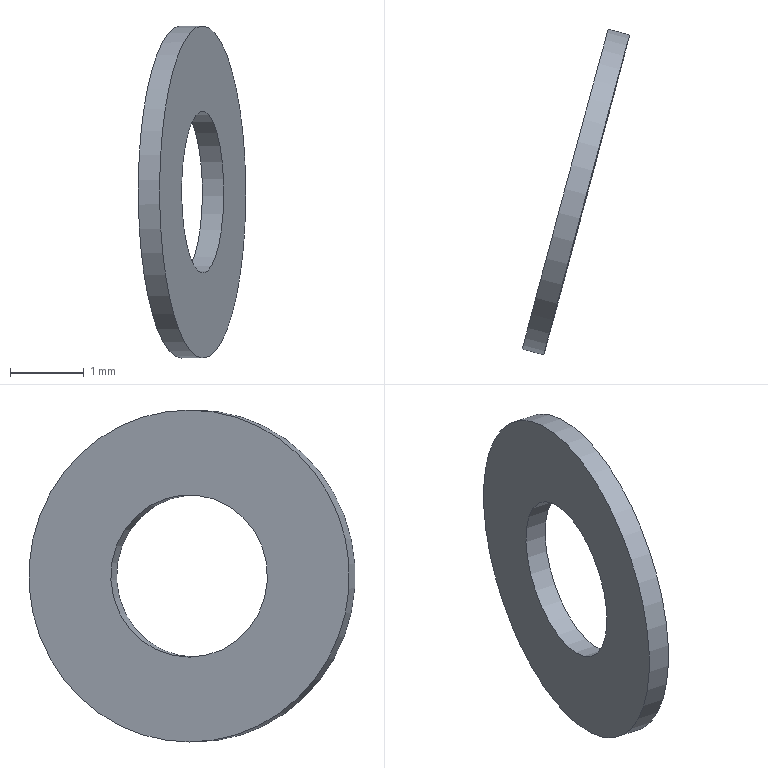Component | NX | GB-T848-2002_M2 | 1 solid | 4 faces | box 1.46 x 4.42 x 4.5 mm | volume 4 mm3 | cylinder 2 | plane 2 | commonest cylinder face diameters 4.5 x1 2.2 x1
STEP:
#1=CARTESIAN_POINT('',(0.,0.,0.));
#2=DIRECTION('',(0.,0.,1.));
#3=DIRECTION('',(1.,0.,0.));
#4=AXIS2_PLACEMENT_3D('',#1,#2,#3);
#5=CARTESIAN_POINT('',(52.266,-56.588,80.689));
#6=VERTEX_POINT('',#5);
#7=CARTESIAN_POINT('',(52.262,-56.588,82.939));
#8=DIRECTION('',(0.9657,-0.2595,0.001964));
#9=DIRECTION('',(0.002034,0.,-1.));
#10=AXIS2_PLACEMENT_3D('',#7,#8,#9);
#11=CIRCLE('',#10,2.25);
#12=CARTESIAN_POINT('',(52.262,-56.588,82.939));
#13=DIRECTION('',(-0.9657,0.2595,-0.001964));
#14=DIRECTION('',(-0.002034,-0.,1.));
#15=AXIS2_PLACEMENT_3D('',#12,#13,#14);
#16=CYLINDRICAL_SURFACE('',#15,2.25);
#17=CARTESIAN_POINT('',(9.425,0.));
#18=DIRECTION('',(-1.,0.));
#19=VECTOR('',#18,1.);
#20=LINE('',#17,#19);
#21=(GEOMETRIC_REPRESENTATION_CONTEXT(2)PARAMETRIC_REPRESENTATION_CONTEXT()REPRESENTATION_CONTEXT('',''));
#22=DEFINITIONAL_REPRESENTATION('',(#20),#21);
#23=PCURVE('',#16,#22);
#24=CARTESIAN_POINT('',(52.262,-56.588,82.939));
#25=DIRECTION('',(0.9657,-0.2595,0.001964));
#26=DIRECTION('',(0.002034,0.,-1.));
#27=AXIS2_PLACEMENT_3D('',#24,#25,#26);
#28=PLANE('',#27);
#29=CARTESIAN_POINT('',(0.,0.));
#30=DIRECTION('',(1.,0.));
#31=AXIS2_PLACEMENT_2D('',#29,#30);
#32=CIRCLE('',#31,2.25);
#33=(GEOMETRIC_REPRESENTATION_CONTEXT(2)PARAMETRIC_REPRESENTATION_CONTEXT()REPRESENTATION_CONTEXT('',''));
#34=DEFINITIONAL_REPRESENTATION('',(#32),#33);
#35=PCURVE('',#28,#34);
#36=SURFACE_CURVE('',#11,(#23,#35),.PCURVE_S1.);
#37=EDGE_CURVE('',#6,#6,#36,.T.);
#38=ORIENTED_EDGE('',*,*,#37,.F.);
#39=CARTESIAN_POINT('',(51.977,-56.51,80.688));
#40=VERTEX_POINT('',#39);
#41=CARTESIAN_POINT('',(52.266,-56.588,80.689));
#42=CARTESIAN_POINT('',(51.977,-56.51,80.688));
#43=B_SPLINE_CURVE_WITH_KNOTS('',1,(#41,#42),.UNSPECIFIED.,.F.,.F.,(2,2),(0.,0.3),.PIECEWISE_BEZIER_KNOTS.);
#44=CARTESIAN_POINT('',(9.425,0.));
#45=DIRECTION('',(0.,1.));
#46=VECTOR('',#45,1.);
#47=LINE('',#44,#46);
#48=(GEOMETRIC_REPRESENTATION_CONTEXT(2)PARAMETRIC_REPRESENTATION_CONTEXT()REPRESENTATION_CONTEXT('',''));
#49=DEFINITIONAL_REPRESENTATION('',(#47),#48);
#50=PCURVE('',#16,#49);
#51=CARTESIAN_POINT('',(3.142,0.));
#52=DIRECTION('',(0.,1.));
#53=VECTOR('',#52,1.);
#54=LINE('',#51,#53);
#55=(GEOMETRIC_REPRESENTATION_CONTEXT(2)PARAMETRIC_REPRESENTATION_CONTEXT()REPRESENTATION_CONTEXT('',''));
#56=DEFINITIONAL_REPRESENTATION('',(#54),#55);
#57=PCURVE('',#16,#56);
#58=SEAM_CURVE('',#43,(#50,#57),.PCURVE_S1.);
#59=EDGE_CURVE('',#6,#40,#58,.T.);
#60=ORIENTED_EDGE('',*,*,#59,.T.);
#61=CARTESIAN_POINT('',(51.972,-56.51,82.938));
#62=DIRECTION('',(0.9657,-0.2595,0.001964));
#63=DIRECTION('',(0.002034,0.,-1.));
#64=AXIS2_PLACEMENT_3D('',#61,#62,#63);
#65=CIRCLE('',#64,2.25);
#66=CARTESIAN_POINT('',(9.425,0.3));
#67=DIRECTION('',(-1.,0.));
#68=VECTOR('',#67,1.);
#69=LINE('',#66,#68);
#70=(GEOMETRIC_REPRESENTATION_CONTEXT(2)PARAMETRIC_REPRESENTATION_CONTEXT()REPRESENTATION_CONTEXT('',''));
#71=DEFINITIONAL_REPRESENTATION('',(#69),#70);
#72=PCURVE('',#16,#71);
#73=CARTESIAN_POINT('',(51.972,-56.51,82.938));
#74=DIRECTION('',(0.9657,-0.2595,0.001964));
#75=DIRECTION('',(0.002034,0.,-1.));
#76=AXIS2_PLACEMENT_3D('',#73,#74,#75);
#77=PLANE('',#76);
#78=CARTESIAN_POINT('',(0.,0.));
#79=DIRECTION('',(1.,0.));
#80=AXIS2_PLACEMENT_2D('',#78,#79);
#81=CIRCLE('',#80,2.25);
#82=(GEOMETRIC_REPRESENTATION_CONTEXT(2)PARAMETRIC_REPRESENTATION_CONTEXT()REPRESENTATION_CONTEXT('',''));
#83=DEFINITIONAL_REPRESENTATION('',(#81),#82);
#84=PCURVE('',#77,#83);
#85=SURFACE_CURVE('',#65,(#72,#84),.PCURVE_S1.);
#86=EDGE_CURVE('',#40,#40,#85,.T.);
#87=ORIENTED_EDGE('',*,*,#86,.T.);
#88=ORIENTED_EDGE('',*,*,#59,.F.);
#89=EDGE_LOOP('',(#38,#60,#87,#88));
#90=FACE_BOUND('',#89,.T.);
#91=ADVANCED_FACE('',(#90),#16,.T.);
#92=CARTESIAN_POINT('',(52.264,-56.588,81.839));
#93=VERTEX_POINT('',#92);
#94=CARTESIAN_POINT('',(52.262,-56.588,82.939));
#95=DIRECTION('',(0.9657,-0.2595,0.001964));
#96=DIRECTION('',(0.002034,-0.,-1.));
#97=AXIS2_PLACEMENT_3D('',#94,#95,#96);
#98=CIRCLE('',#97,1.1);
#99=CARTESIAN_POINT('',(52.262,-56.588,82.939));
#100=DIRECTION('',(-0.9657,0.2595,-0.001964));
#101=DIRECTION('',(-0.002034,0.,1.));
#102=AXIS2_PLACEMENT_3D('',#99,#100,#101);
#103=CYLINDRICAL_SURFACE('',#102,1.1);
#104=CARTESIAN_POINT('',(9.425,0.));
#105=DIRECTION('',(-1.,0.));
#106=VECTOR('',#105,1.);
#107=LINE('',#104,#106);
#108=(GEOMETRIC_REPRESENTATION_CONTEXT(2)PARAMETRIC_REPRESENTATION_CONTEXT()REPRESENTATION_CONTEXT('',''));
#109=DEFINITIONAL_REPRESENTATION('',(#107),#108);
#110=PCURVE('',#103,#109);
#111=CARTESIAN_POINT('',(0.,0.));
#112=DIRECTION('',(1.,-0.));
#113=AXIS2_PLACEMENT_2D('',#111,#112);
#114=CIRCLE('',#113,1.1);
#115=(GEOMETRIC_REPRESENTATION_CONTEXT(2)PARAMETRIC_REPRESENTATION_CONTEXT()REPRESENTATION_CONTEXT('',''));
#116=DEFINITIONAL_REPRESENTATION('',(#114),#115);
#117=PCURVE('',#28,#116);
#118=SURFACE_CURVE('',#98,(#110,#117),.PCURVE_S1.);
#119=EDGE_CURVE('',#93,#93,#118,.T.);
#120=ORIENTED_EDGE('',*,*,#119,.F.);
#121=CARTESIAN_POINT('',(51.974,-56.51,81.838));
#122=VERTEX_POINT('',#121);
#123=CARTESIAN_POINT('',(52.264,-56.588,81.839));
#124=CARTESIAN_POINT('',(51.974,-56.51,81.838));
#125=B_SPLINE_CURVE_WITH_KNOTS('',1,(#123,#124),.UNSPECIFIED.,.F.,.F.,(2,2),(0.,0.3),.PIECEWISE_BEZIER_KNOTS.);
#126=CARTESIAN_POINT('',(9.425,0.));
#127=DIRECTION('',(0.,1.));
#128=VECTOR('',#127,1.);
#129=LINE('',#126,#128);
#130=(GEOMETRIC_REPRESENTATION_CONTEXT(2)PARAMETRIC_REPRESENTATION_CONTEXT()REPRESENTATION_CONTEXT('',''));
#131=DEFINITIONAL_REPRESENTATION('',(#129),#130);
#132=PCURVE('',#103,#131);
#133=CARTESIAN_POINT('',(3.142,0.));
#134=DIRECTION('',(0.,1.));
#135=VECTOR('',#134,1.);
#136=LINE('',#133,#135);
#137=(GEOMETRIC_REPRESENTATION_CONTEXT(2)PARAMETRIC_REPRESENTATION_CONTEXT()REPRESENTATION_CONTEXT('',''));
#138=DEFINITIONAL_REPRESENTATION('',(#136),#137);
#139=PCURVE('',#103,#138);
#140=SEAM_CURVE('',#125,(#132,#139),.PCURVE_S1.);
#141=EDGE_CURVE('',#93,#122,#140,.T.);
#142=ORIENTED_EDGE('',*,*,#141,.T.);
#143=CARTESIAN_POINT('',(51.972,-56.51,82.938));
#144=DIRECTION('',(0.9657,-0.2595,0.001964));
#145=DIRECTION('',(0.002034,-0.,-1.));
#146=AXIS2_PLACEMENT_3D('',#143,#144,#145);
#147=CIRCLE('',#146,1.1);
#148=CARTESIAN_POINT('',(9.425,0.3));
#149=DIRECTION('',(-1.,0.));
#150=VECTOR('',#149,1.);
#151=LINE('',#148,#150);
#152=(GEOMETRIC_REPRESENTATION_CONTEXT(2)PARAMETRIC_REPRESENTATION_CONTEXT()REPRESENTATION_CONTEXT('',''));
#153=DEFINITIONAL_REPRESENTATION('',(#151),#152);
#154=PCURVE('',#103,#153);
#155=CARTESIAN_POINT('',(0.,0.));
#156=DIRECTION('',(1.,-0.));
#157=AXIS2_PLACEMENT_2D('',#155,#156);
#158=CIRCLE('',#157,1.1);
#159=(GEOMETRIC_REPRESENTATION_CONTEXT(2)PARAMETRIC_REPRESENTATION_CONTEXT()REPRESENTATION_CONTEXT('',''));
#160=DEFINITIONAL_REPRESENTATION('',(#158),#159);
#161=PCURVE('',#77,#160);
#162=SURFACE_CURVE('',#147,(#154,#161),.PCURVE_S1.);
#163=EDGE_CURVE('',#122,#122,#162,.T.);
#164=ORIENTED_EDGE('',*,*,#163,.T.);
#165=ORIENTED_EDGE('',*,*,#141,.F.);
#166=EDGE_LOOP('',(#120,#142,#164,#165));
#167=FACE_BOUND('',#166,.F.);
#168=ADVANCED_FACE('',(#167),#103,.F.);
#169=ORIENTED_EDGE('',*,*,#37,.T.);
#170=EDGE_LOOP('',(#169));
#171=FACE_BOUND('',#170,.T.);
#172=ORIENTED_EDGE('',*,*,#119,.F.);
#173=EDGE_LOOP('',(#172));
#174=FACE_BOUND('',#173,.T.);
#175=ADVANCED_FACE('',(#171,#174),#28,.T.);
#176=ORIENTED_EDGE('',*,*,#86,.F.);
#177=EDGE_LOOP('',(#176));
#178=FACE_BOUND('',#177,.T.);
#179=ORIENTED_EDGE('',*,*,#163,.T.);
#180=EDGE_LOOP('',(#179));
#181=FACE_BOUND('',#180,.T.);
#182=ADVANCED_FACE('',(#178,#181),#77,.F.);
#183=CLOSED_SHELL('',(#91,#168,#175,#182));
#184=MANIFOLD_SOLID_BREP('',#183);
#185=(LENGTH_UNIT()NAMED_UNIT(*)SI_UNIT(.MILLI.,.METRE.));
#186=UNCERTAINTY_MEASURE_WITH_UNIT(LENGTH_MEASURE(0.00001),#185,'','');
#187=(NAMED_UNIT(*)PLANE_ANGLE_UNIT()SI_UNIT($,.RADIAN.));
#188=(NAMED_UNIT(*)SI_UNIT($,.STERADIAN.)SOLID_ANGLE_UNIT());
#189=(GEOMETRIC_REPRESENTATION_CONTEXT(3)GLOBAL_UNCERTAINTY_ASSIGNED_CONTEXT((#186))GLOBAL_UNIT_ASSIGNED_CONTEXT((#185,#187,#188))REPRESENTATION_CONTEXT('',''));
#190=ADVANCED_BREP_SHAPE_REPRESENTATION('',(#4,#184),#189);